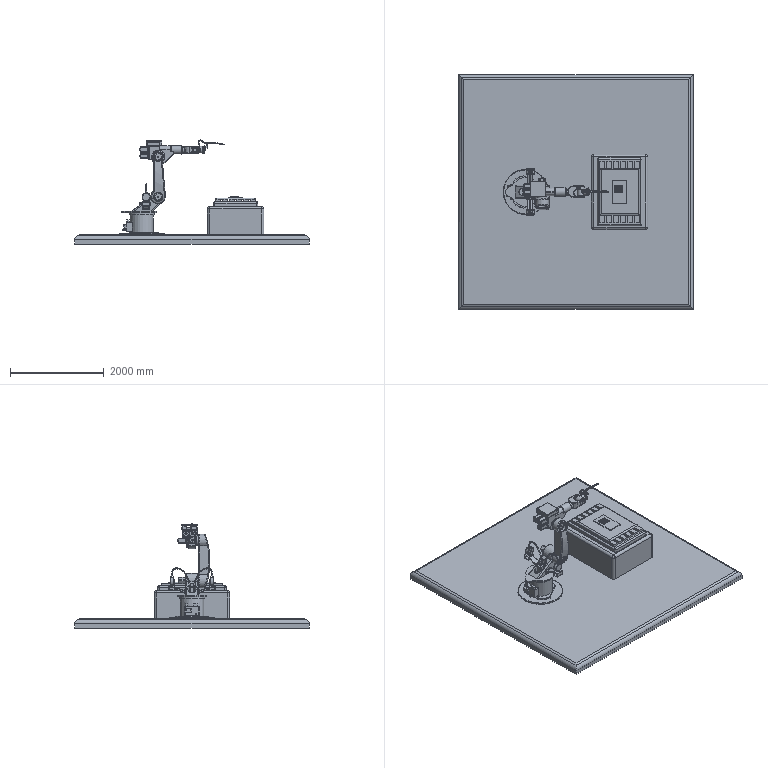Assembly | NX | mm | 16 component files | 241 solids | 2877 faces | box 5000 x 5000 x 2217.82 mm | volume 6577921366 mm3 | plane 1942 | cylinder 607 | sphere 121 | torus 83 | spline 54 | cone 41 | other 29 | commonest cylinder face diameters 10 x244 4 x138 20 x61 6 x36 16 x27 180 x12 60 x12 1 x12
Bill of materials:
unnamed part 1 | 1 |  | Rectangular block-shaped body with rounded vertical edges and a stepped top: a smaller raised tier, then a top plate with a shallow rectangular raised pad. A row of small rectangular tabs runs along each of the two long edges of the upper tier.
unnamed part 2 | 1 |  | Upright cylinder with a slightly larger top lip, standing on a thin round base disc. A raised irregular polygonal pad sits between the cylinder and the disc, and a cluster of small rectangular blocks sticks out from one side of the cylinder.
unnamed part 3 | 1 |  | Long, slender rectangular bar or strip with a plain rectangular cross-section.
unnamed part 4 | 1 |  | Thin, flat, square plate with sharp edges and no visible features.
unnamed part 5 | 1 |  | Clip or clamp-like body with an open C-shaped jaw (U-slot) and a rounded closed end. A short cylindrical boss sticks out from the back, and the side faces carry rows of small raised hexagonal dots.
unnamed part 6 | 1 |  | Elbow-shaped solid made of two short, rounded cylindrical sections meeting at a right angle. Each flat end face has a small central hole, and a thin disc or collar sits at one end.
unnamed part 7 | 1 |  | Thin, flat, square plate with a small chamfer or bevel around the top edges.
unnamed part 8 | 1 |  | Complex multi-feature body on a thin, roughly circular base plate. It has a central drum-shaped housing, two side arms ending in round cylindrical pods, arched curved rods linking the pods to the central body, and a rectangular block with an opening on one side.
unnamed part 9 | 1 |  | Long, slender, paired tubular member with a hook-shaped curved end at one side and two thin pin-like tips at the other. A small bracket with a round flanged disc hangs below it.
unnamed part 10 | 1 |  | Compact multi-block body: a rectangular central block with a stepped cylindrical shaft extending to one side, a short round boss on another face, two parallel rectangular prongs on the opposite side, and a shallow rectangular open-top tray-like box on top.
unnamed part 11 | 5 |  | Plain rectangular solid block (cuboid) with sharp edges.
unnamed part 12 | 1 |  | Link- or lever-shaped arm with a rounded circular boss at each end, joined by a slightly tapered and curved web. Each boss face has a shallow recess with a ring of small dots.
Mates:
1. fix | 1_BASE 1 component
2. fix | 9_FLOOR 1 component
3. touch align | 2_SHOULDER_ROTATOR 1 face | 1_BASE 1 face
4. concentric | 2_SHOULDER_ROTATOR 1 edge | 1_BASE 1 edge
5. touch align | 2_SHOULDER_ROTATOR 1 face | 3_SHOULDER 1 face
6. concentric | 2_SHOULDER_ROTATOR 1 edge | 3_SHOULDER 1 edge
7. touch align | 4_ELBOW_PIVOT 1 face | 3_SHOULDER 1 face
8. concentric | 4_ELBOW_PIVOT 1 edge | 3_SHOULDER 1 edge
9. touch align | 5_FOREARM 1 face | 4_ELBOW_PIVOT 1 face
10. concentric | 4_ELBOW_PIVOT 1 edge | 5_FOREARM 1 edge
11. touch align | 5_FOREARM 1 face | 6_WRIST 1 face
12. concentric | 6_WRIST 1 edge | 5_FOREARM 1 edge
13. touch align | 6_WRIST 1 face | 7_NOZZLE 1 face
14. concentric | 7_NOZZLE 1 edge | 6_WRIST 1 edge
15. fix | 8_WORKBENCH 1 component
16. fix | 10_WORKPIECE 1 component
17. fix | 11_OBJECT 5 component
18. fix | 11_OBJECT 4 component
19. fix | 11_OBJECT 3 component
20. fix | 11_OBJECT 2 component
21. fix | 11_OBJECT 1 component
22. fix | 12_SINKBODY 1 component